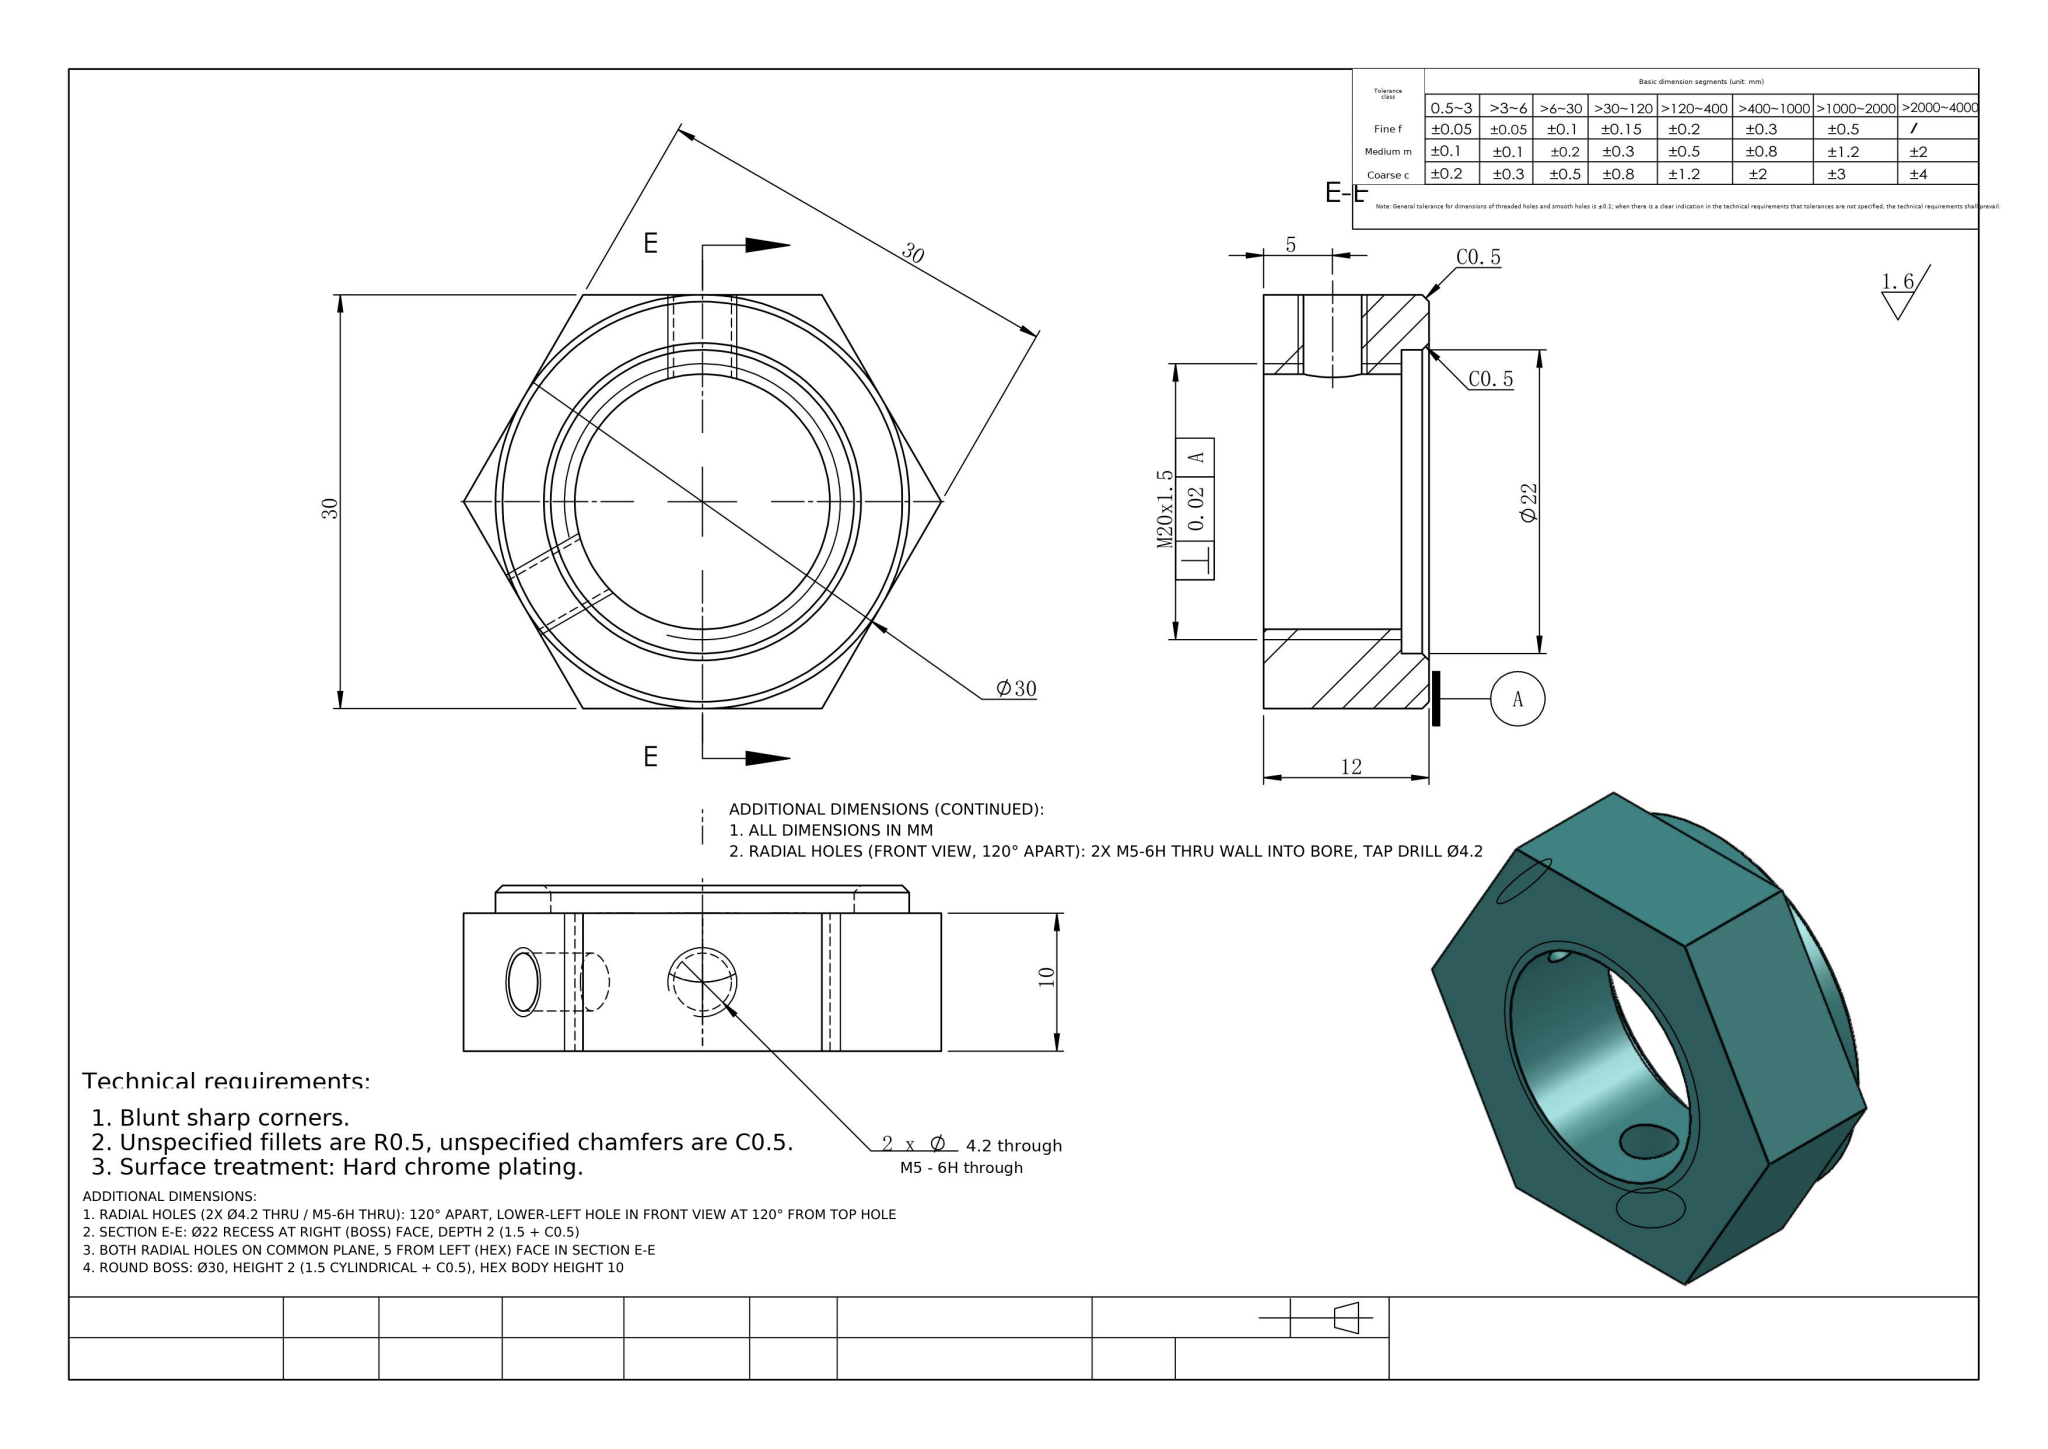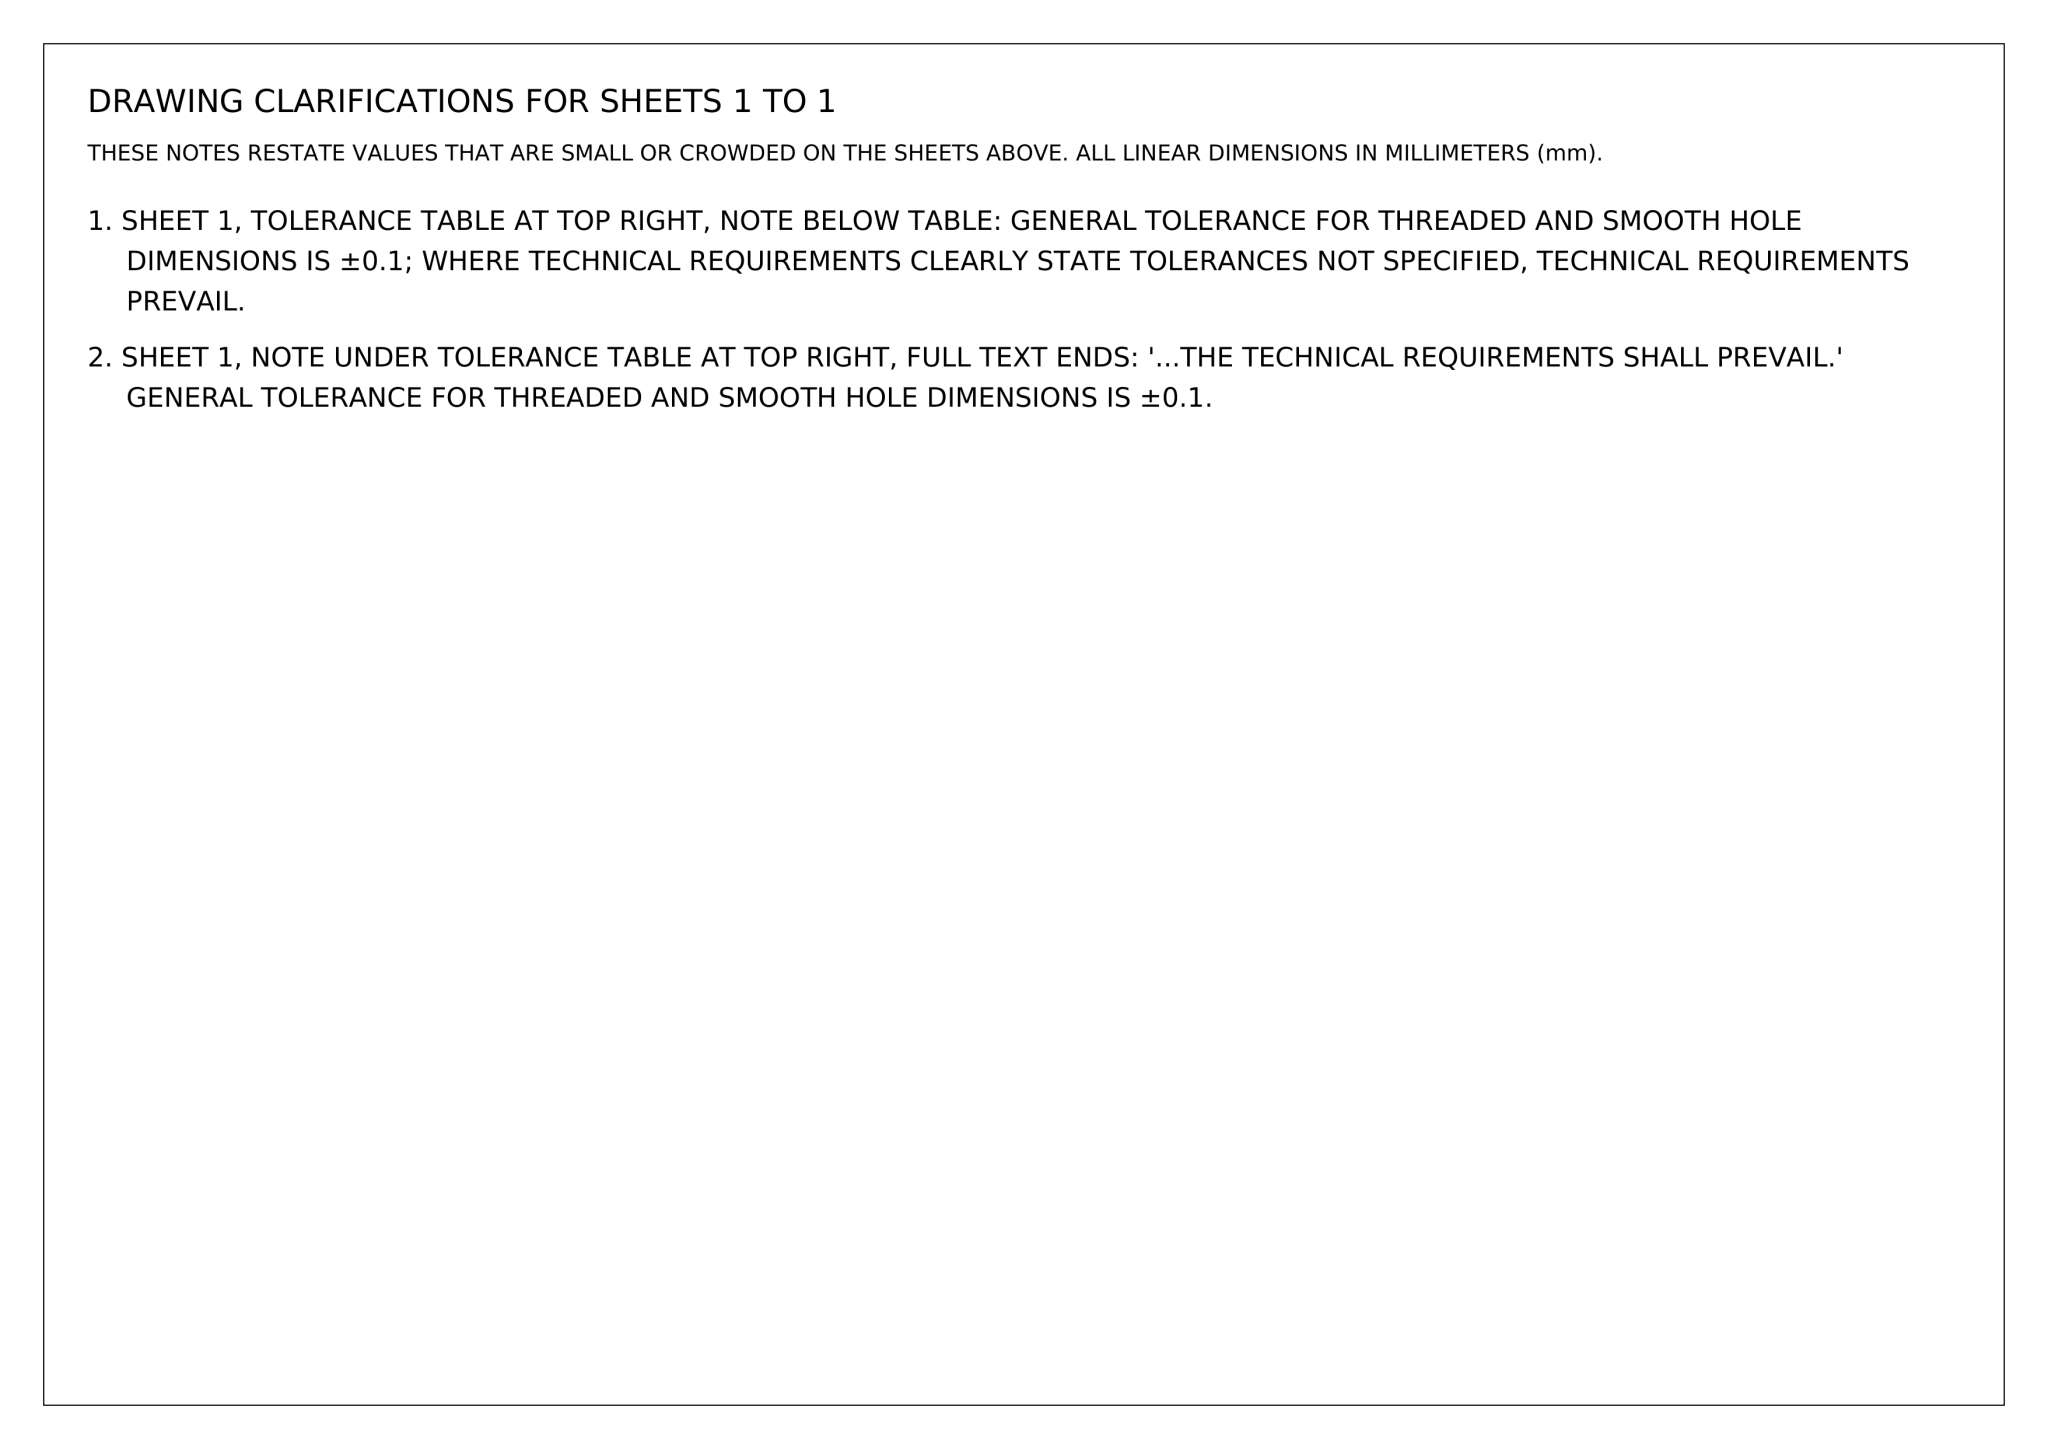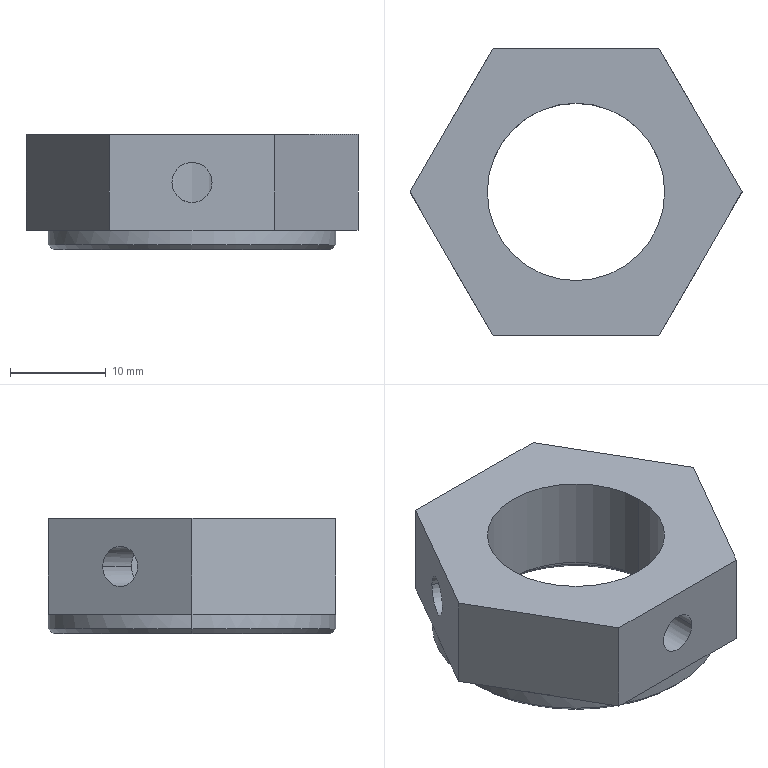Part | NX | mm | 1 solid | 29 faces | box 34.64 x 30 x 12 mm | volume 5578 mm3 | plane 15 | cylinder 10 | cone 4 | commonest cylinder face diameters 4.2 x4 22 x2 30 x2 18.5 x2